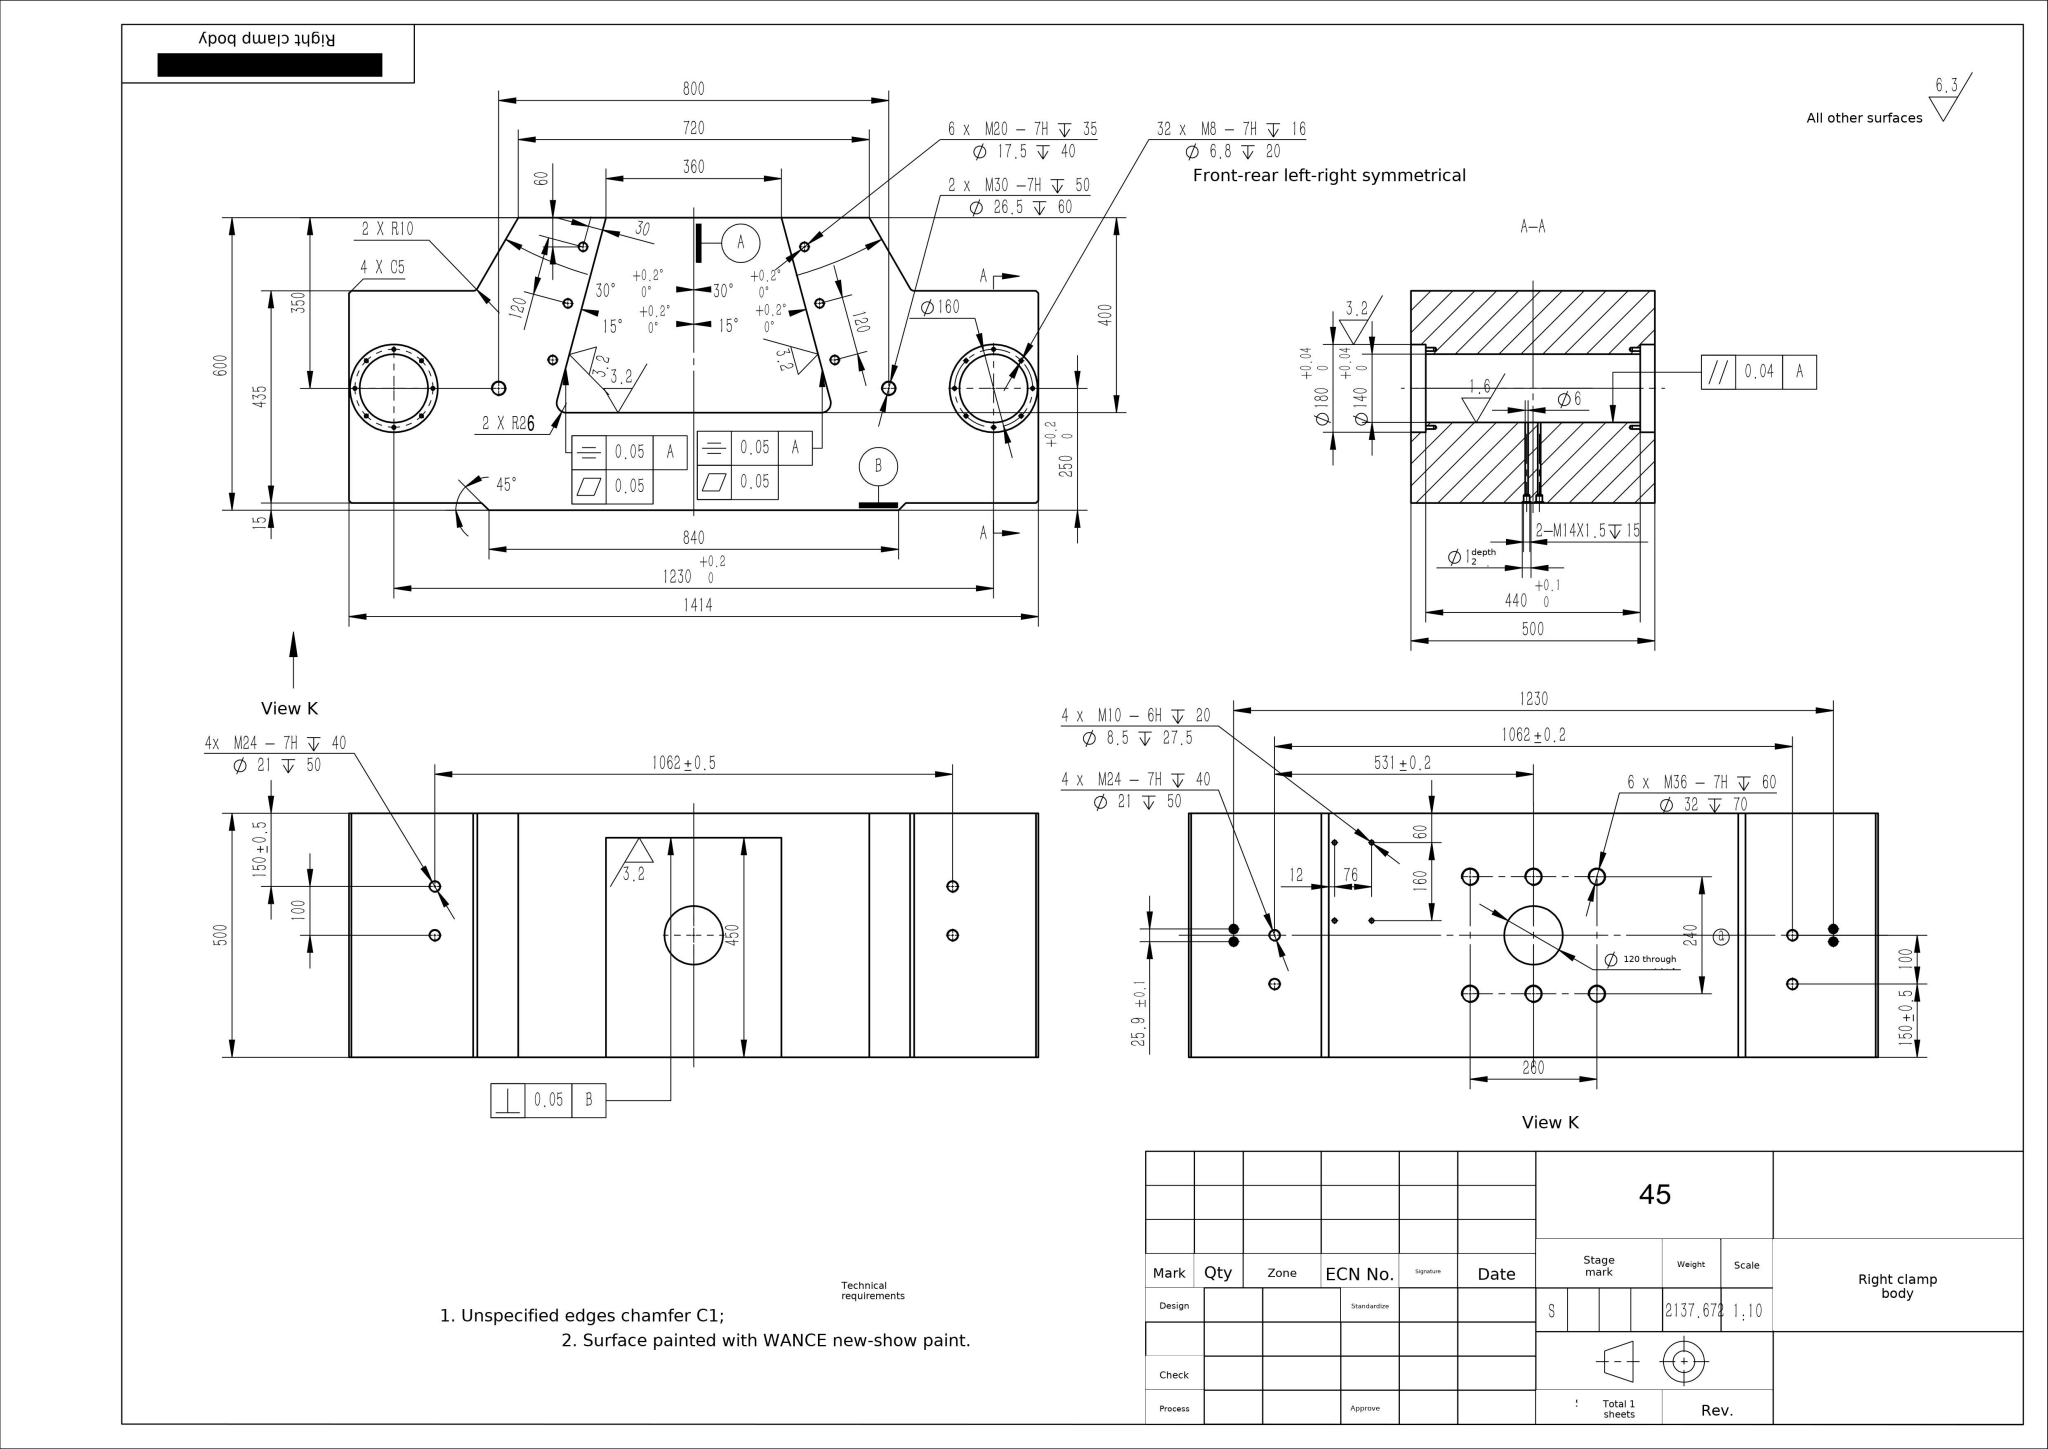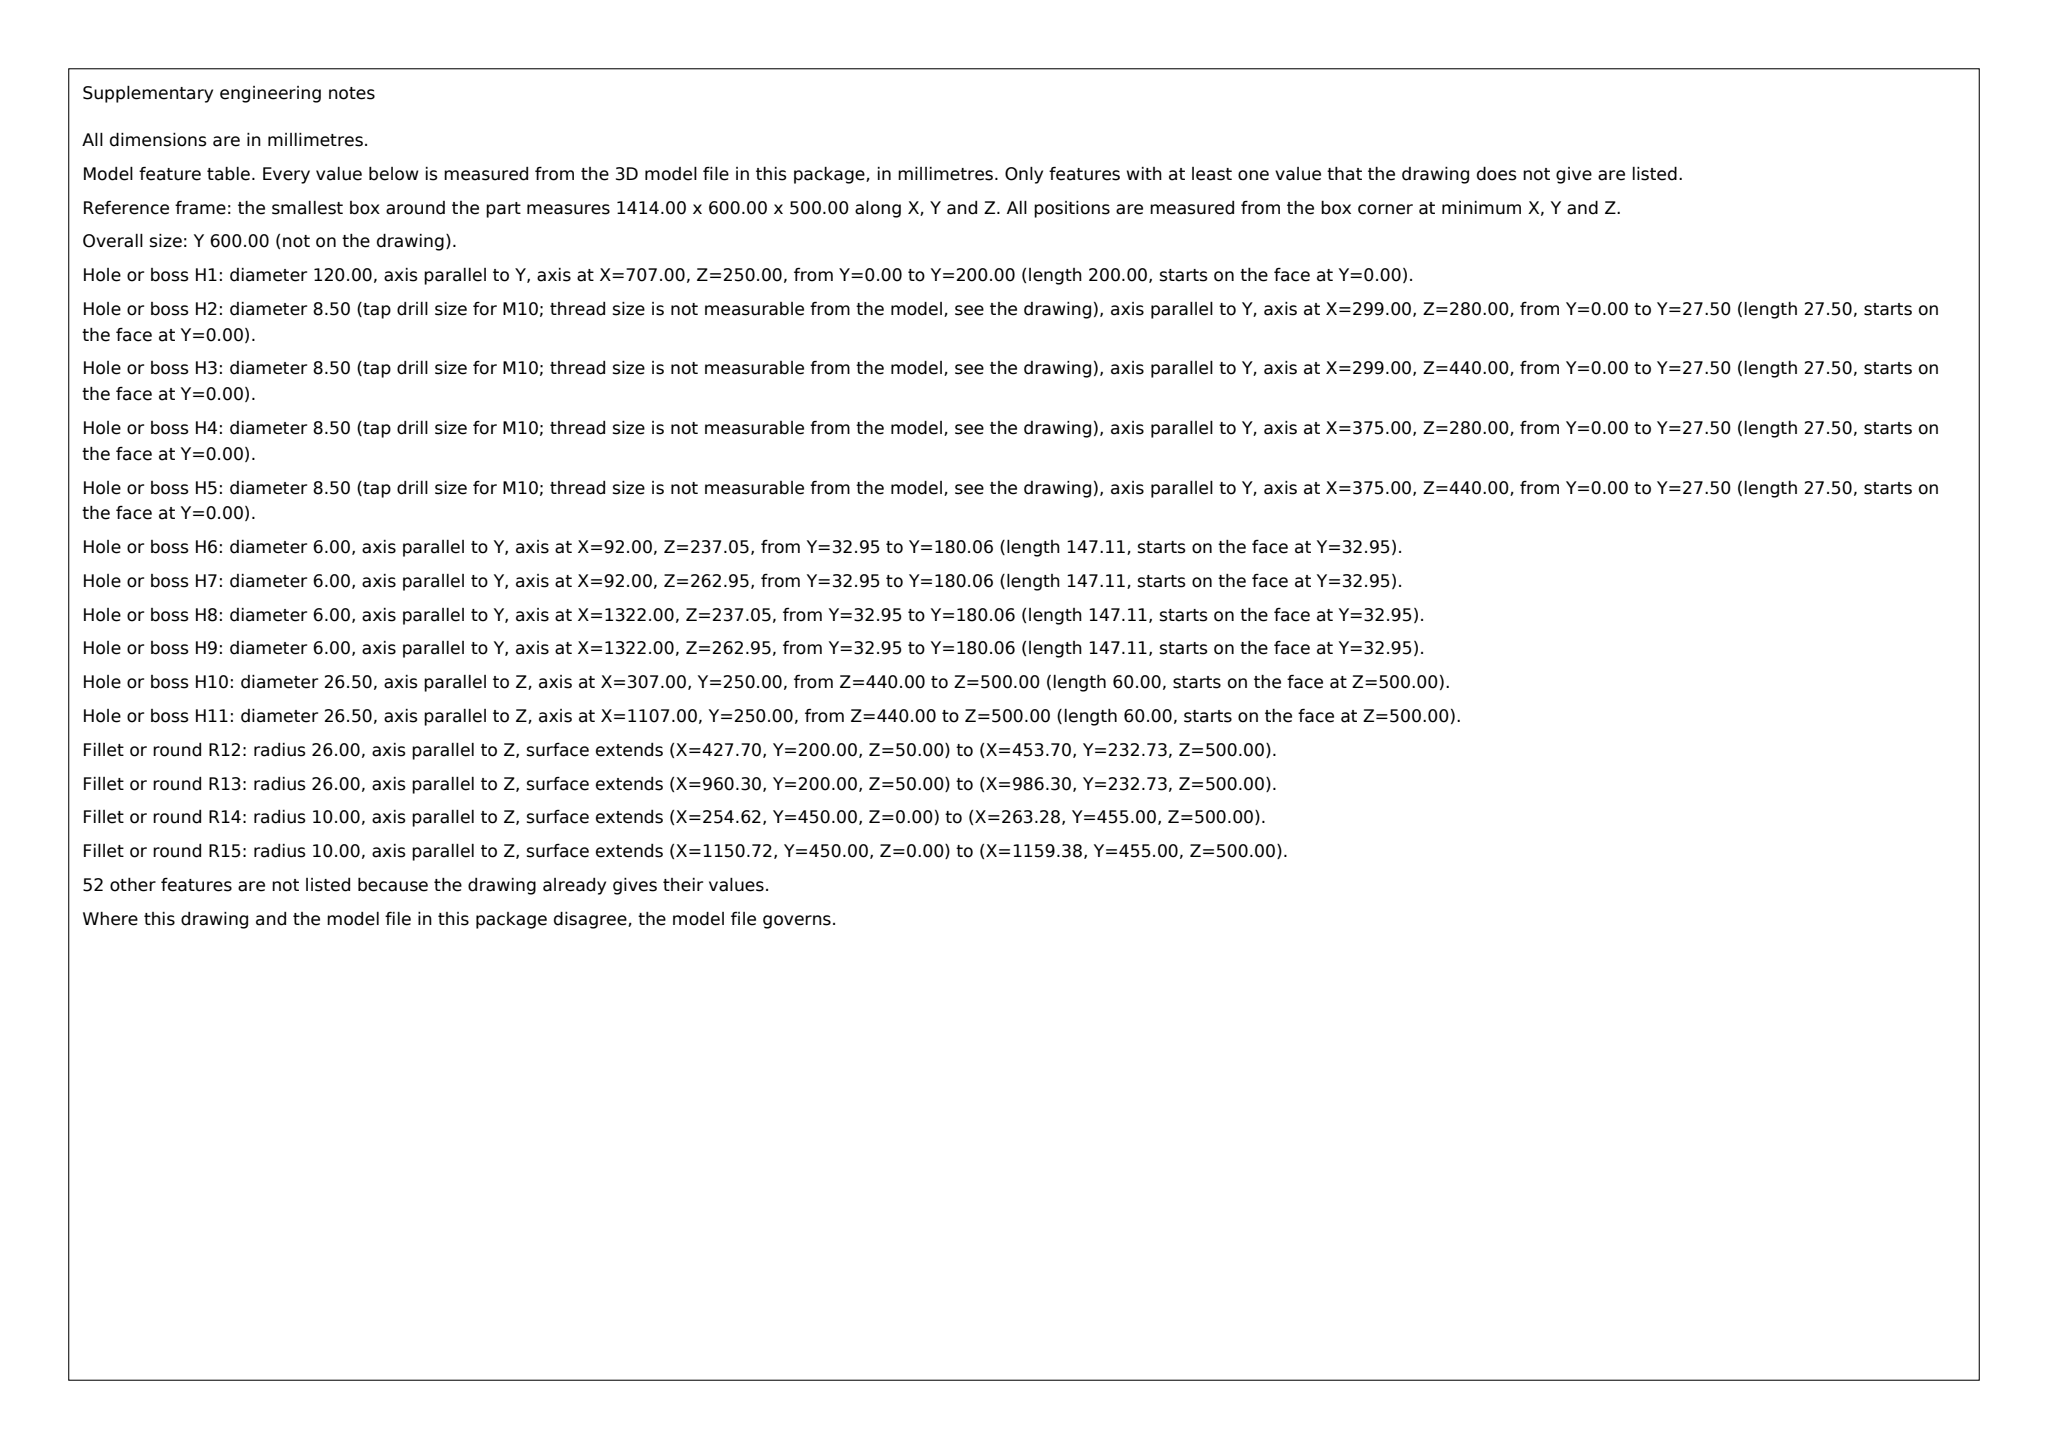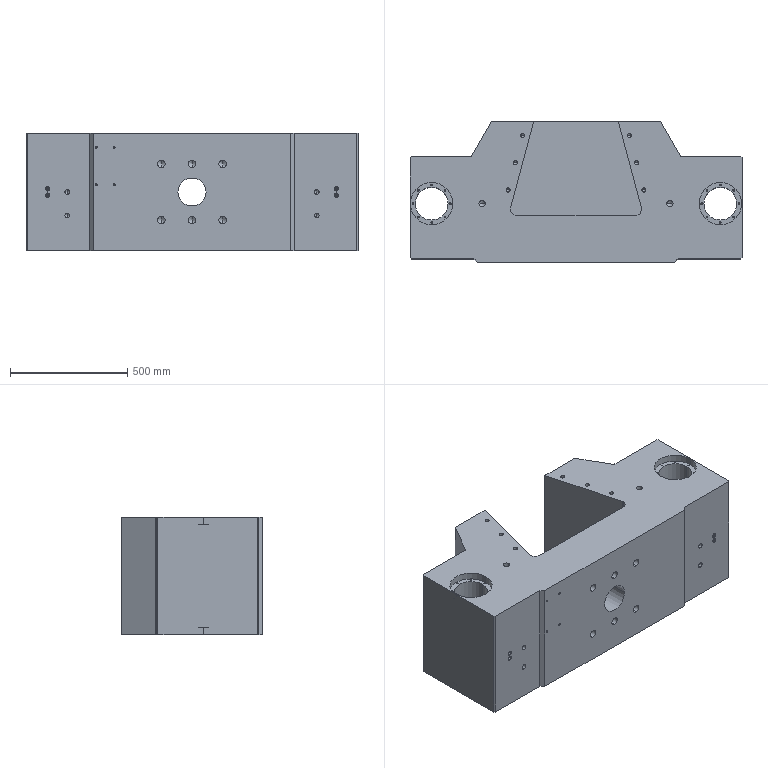Part | SolidWorks | mm | 1 solid | 313 faces | box 1414 x 600 x 500 mm | volume 271030464 mm3 | cylinder 159 | cone 124 | plane 30 | commonest cylinder face diameters 6.8 x64 21 x16 32 x12 17.5 x12 8.5 x8 6 x8 12.5 x8 18 x8